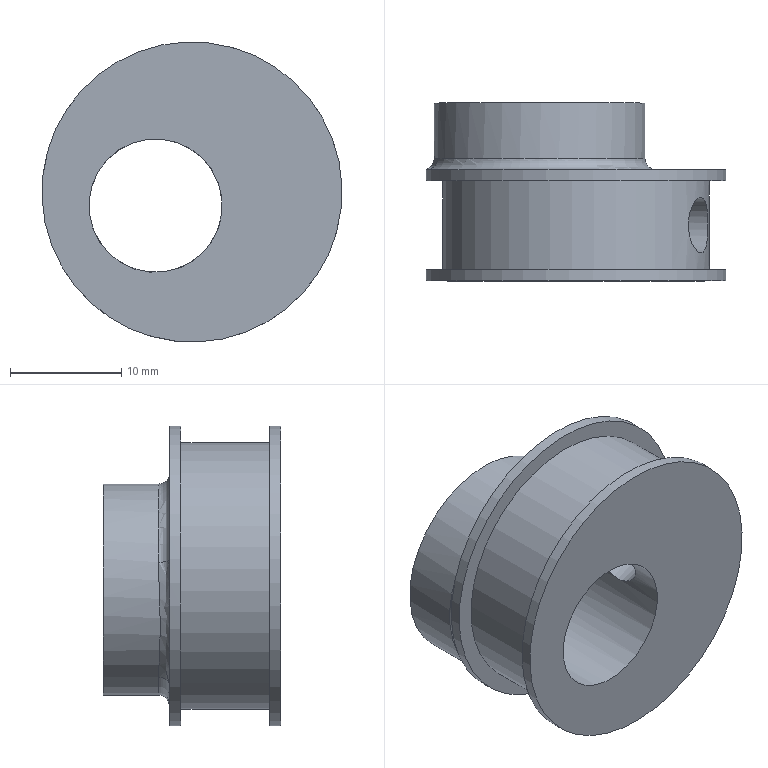Component | NX | ECCENTRIC_SHAFT | 1 solid | 13 faces | volume 4480 mm3 | cylinder 6 | plane 5 | torus 1 | spline 1 | commonest cylinder face diameters 27 x2 24 x1 19 x1 12 x1 5 x1